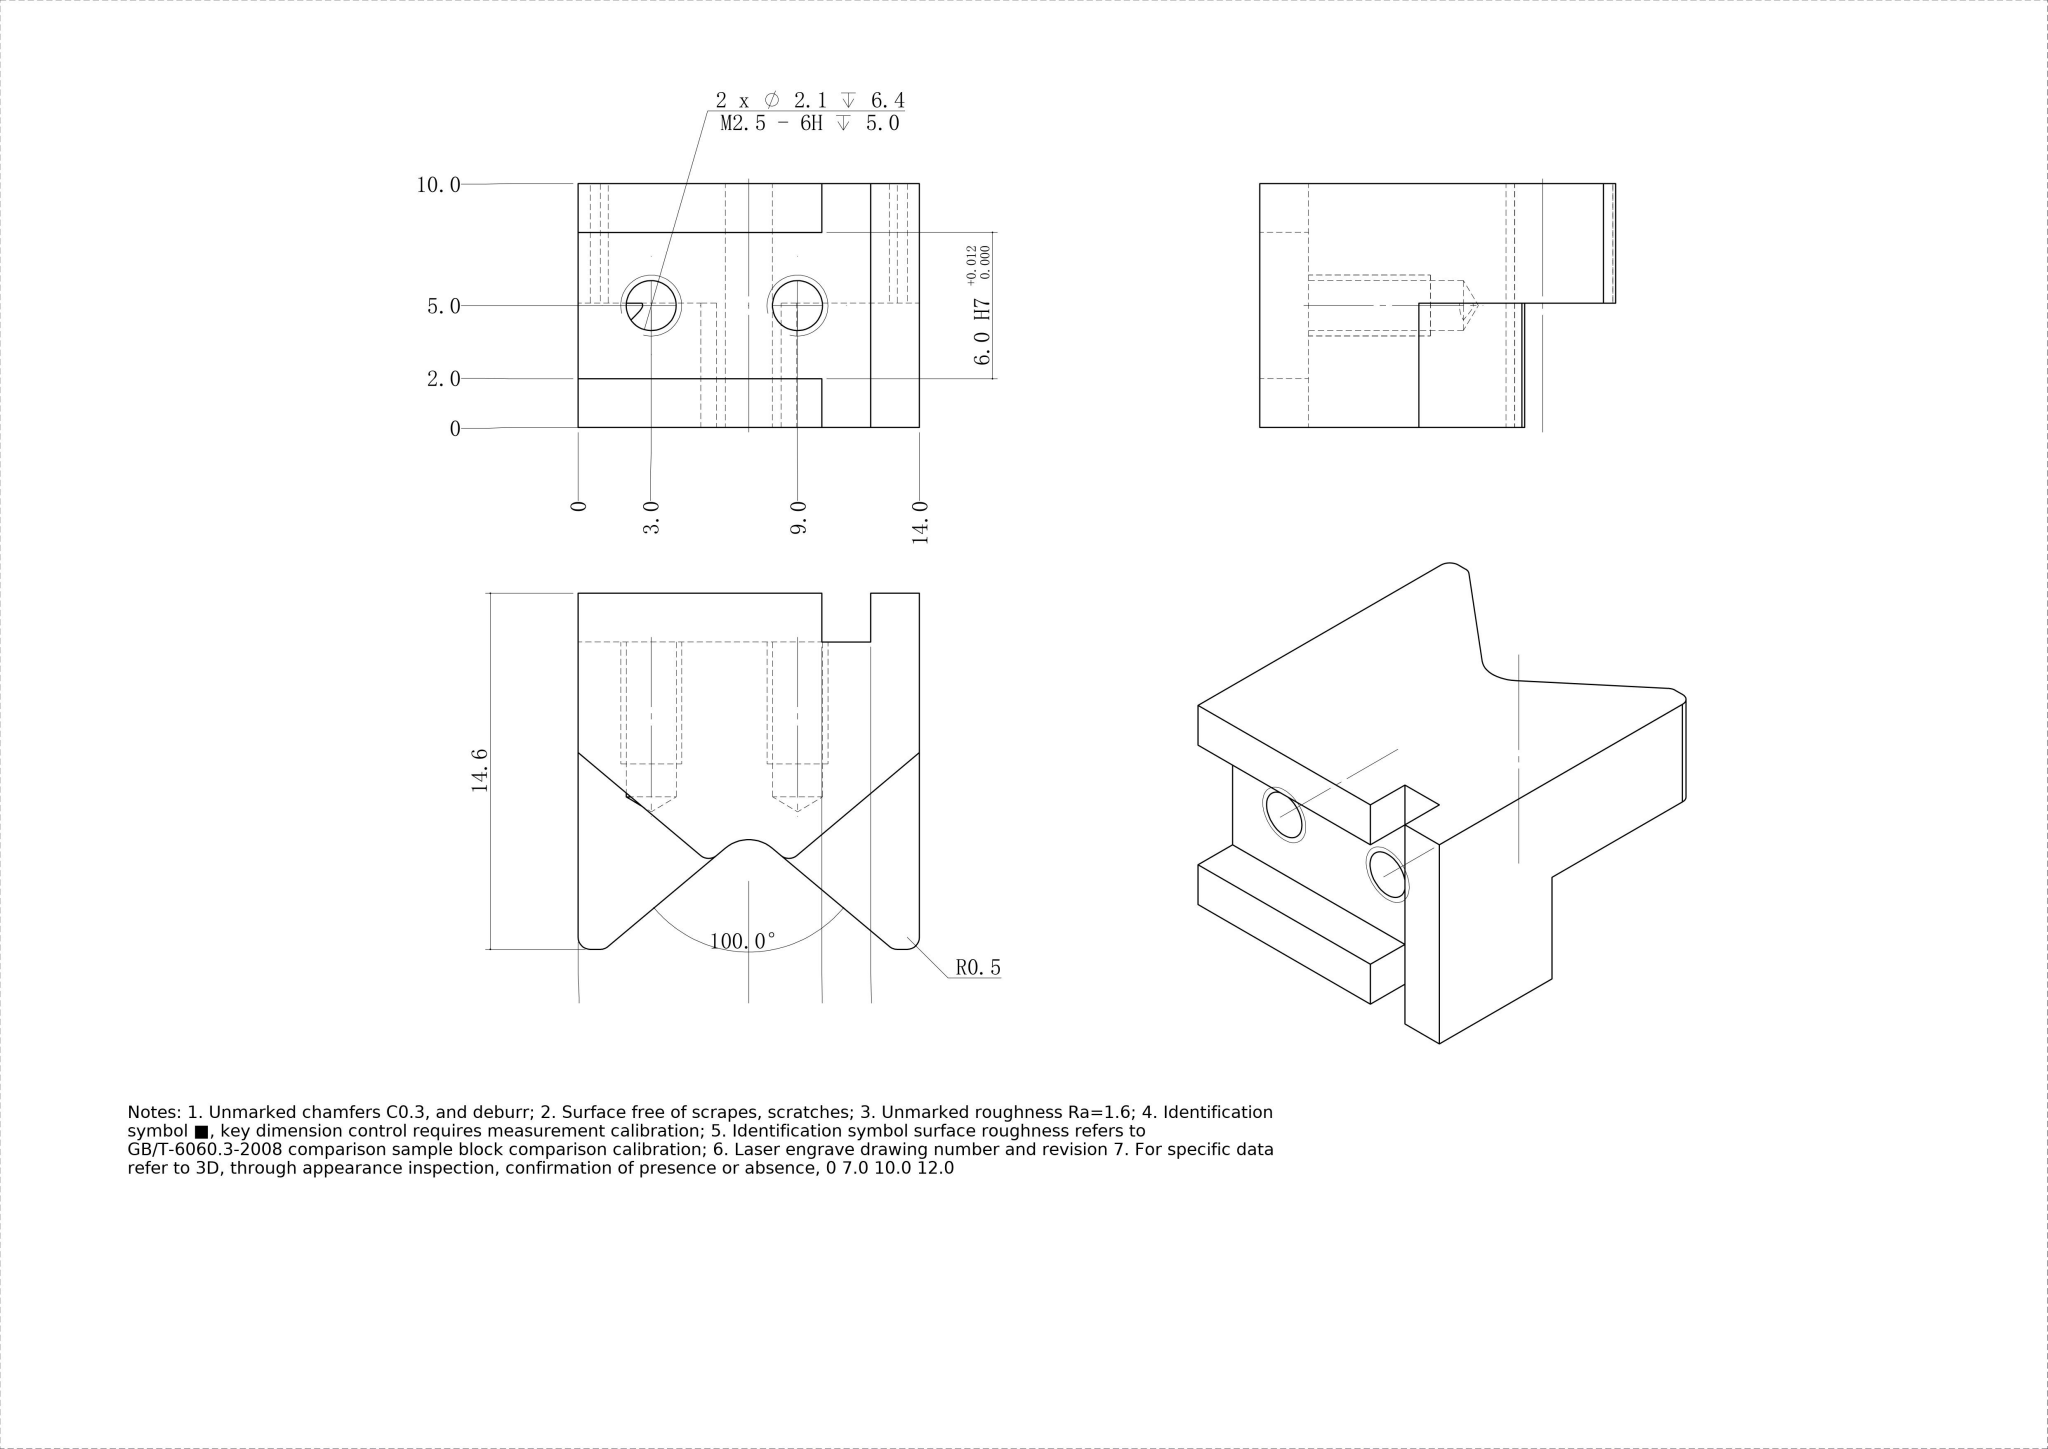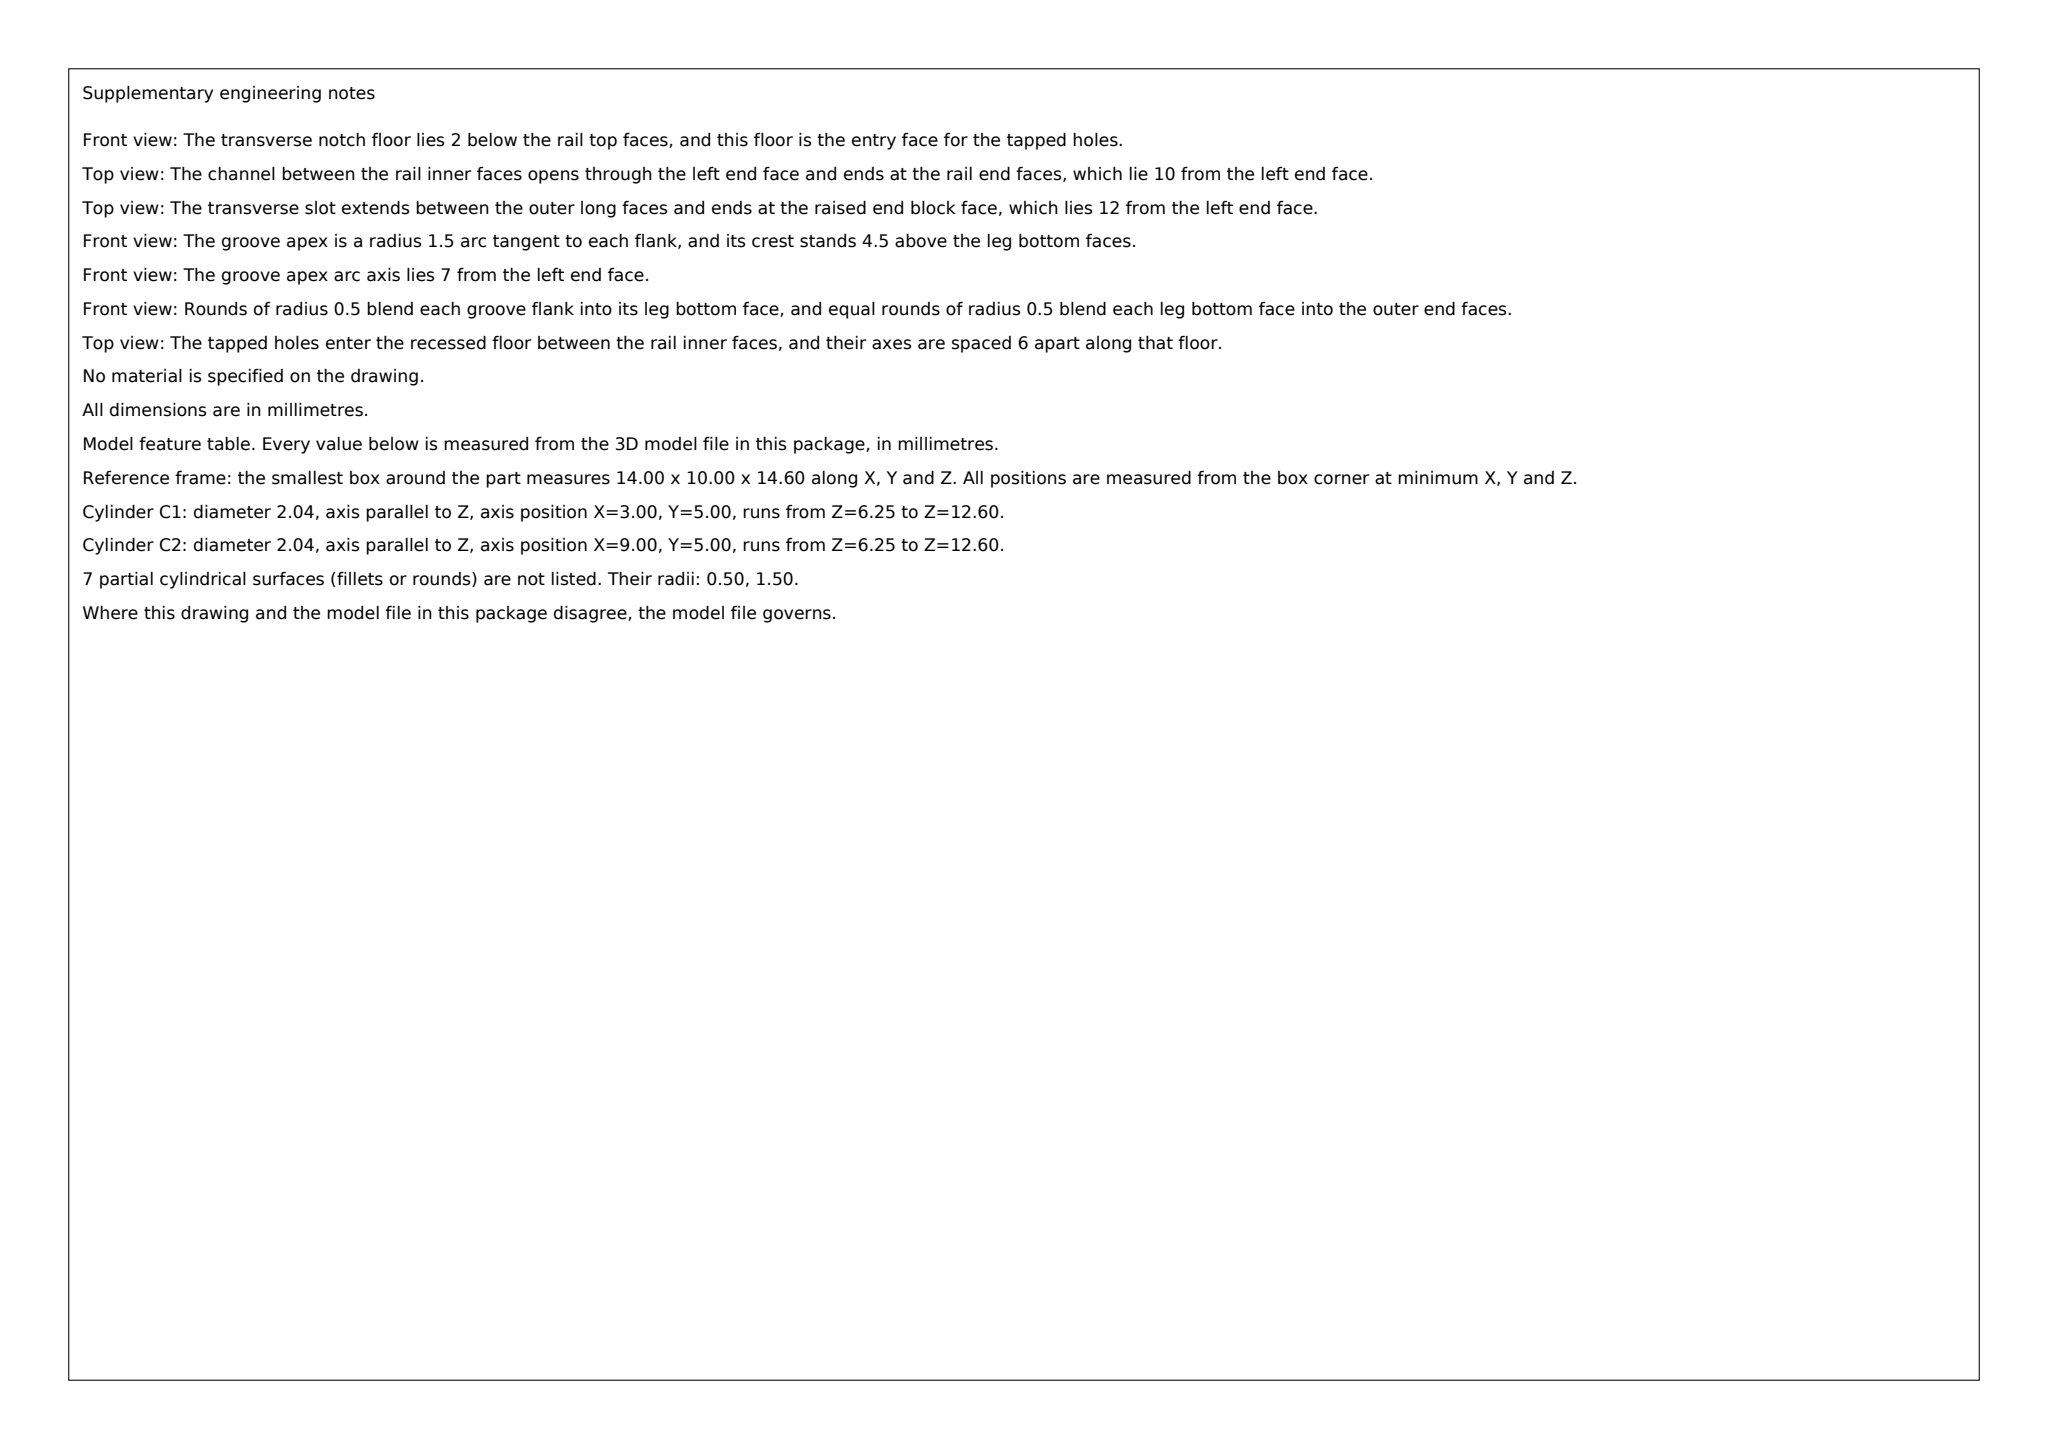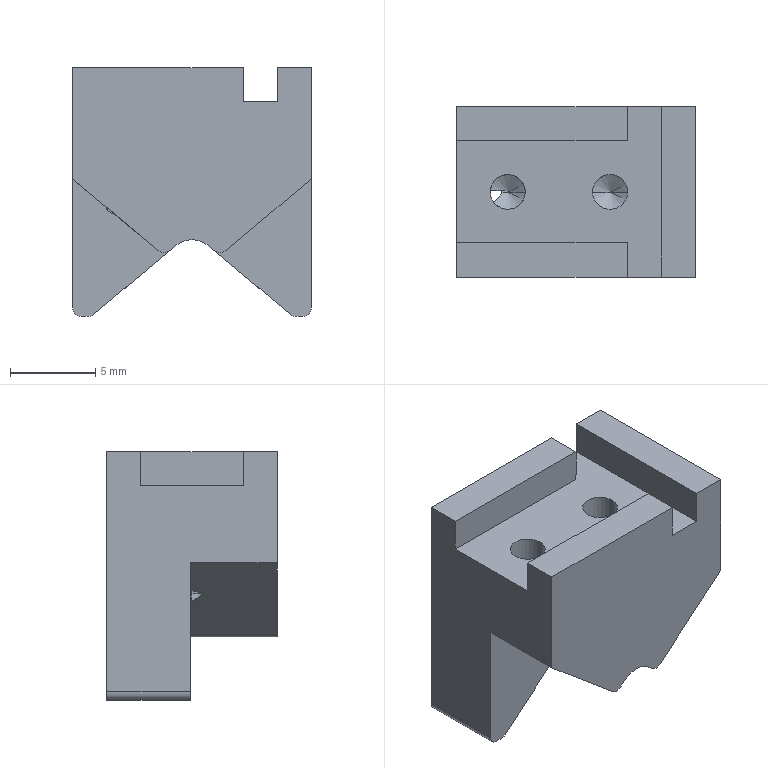Part | SolidWorks | mm | 1 solid | 38 faces | box 14 x 10 x 14.6 mm | volume 1310 mm3 | plane 21 | cylinder 13 | cone 4 | commonest cylinder face diameters 1 x8 2.05 x4 3 x1
Drawing notes:
FRONT VIEW: V-GROOVE / R1.5 CL AT X=7.0 FROM LH END FACE | from the solid: Ø3.0 y-axis cyl at x=7.0, z=3.0; V form centred on same axis
STEP / SHOULDER FACE 10.0 FROM LH END FACE | from the solid: axis_plane normal x, offset 10.0 (count 2)
TOP NOTCH 2.0 DP x 2.0 WIDE; FACE 12.0 FROM LH END FACE | from the solid: x planes at 12.0 and 14.0 (bbox X=14.0); notch depth 2.0 (balloon 1)
SIDE VIEW: RH STEP 2.0 DP; FACE 8.0 FROM FRONT FACE Y=0 | from the solid: y planes at 8.0 and 10.0; bbox Y=10.0
V-GROOVE RUN-OUT FACE 5.1 FROM FRONT FACE Y=0 | from the solid: axis_plane normal y, offset 5.1 (count 2); Ø1.0 y-cyl length 5.1
build123d program:
from build123d import *

# Parameters (mm, degrees)
SKETCH1_2_W             = 14
SKETCH1_2_H             = 10
BOSS_EXTRUDE1_DEPTH     = 7.3
CUT_EXTRUDE2_DEPTH      = 15.223
SKETCH1_W               = 24
SKETCH1_H               = 6
EXTRUDE1_DEPTH          = 2
SKETCH2_W               = 2
SKETCH2_H               = 10
EXTRUDE2_DEPTH          = 2
EXTRUDE3_DEPTH          = 5.1
M2_5_TAPPED_HOLE1_D     = 2.05
M2_5_TAPPED_HOLE1_DEPTH = 6.35
M2_5_TAPPED_HOLE1_TIP   = 0.6159
FILLET1_R               = 0.5


with BuildPart() as part:
    # Sketch1_2 → Boss-Extrude1 (new, symmetric)
    with BuildSketch(Plane.XY):
        Rectangle(SKETCH1_2_W, SKETCH1_2_H)
    extrude(amount=BOSS_EXTRUDE1_DEPTH, both=True)

    # Sketch4 → Cut-Extrude2 (cut, through all)
    with BuildSketch(Plane(origin=(0, -5, 0), x_dir=(-1, 0, 0), z_dir=(0, -1, 0))):
        with BuildLine():
            Line((-5.909, 7.3), (-0.9642, 3.151))
            ThreePointArc((-0.9642, 3.151), (0, 2.8), (0.9642, 3.151))
            Line((0.9642, 3.151), (5.909, 7.3))
            Line((5.909, 7.3), (-5.909, 7.3))
        make_face()
    extrude(amount=-CUT_EXTRUDE2_DEPTH, mode=Mode.SUBTRACT)

    # Sketch1 → Extrude1 (cut)
    with BuildSketch(Plane(origin=(0, 0, 7.3), x_dir=(-1, 0, 0), z_dir=(0, 0, -1))):
        with Locations((7, 0)):
            Rectangle(SKETCH1_W, SKETCH1_H)
    extrude(amount=EXTRUDE1_DEPTH, mode=Mode.SUBTRACT)

    # Sketch2 → Extrude2 (cut)
    with BuildSketch(Plane(origin=(0, 0, 7.3), x_dir=(-1, 0, 0), z_dir=(0, 0, -1))):
        with Locations((-4, 0)):
            Rectangle(SKETCH2_W, SKETCH2_H)
    extrude(amount=EXTRUDE2_DEPTH, mode=Mode.SUBTRACT)

    # Sketch3 → Extrude3 (cut)
    with BuildSketch(Plane.XZ.offset(5)):
        Polygon((7, -7.3), (7, 0.7683), (1.647, -3.724), (5.909, -7.3), align=None)
        Polygon((-5.909, -7.3), (-1.647, -3.724), (-7, 0.7683), (-7, -7.3), align=None)
    extrude(amount=-EXTRUDE3_DEPTH, mode=Mode.SUBTRACT)

    # M2.5 Tapped Hole1
    with Locations(Plane.XY.offset(5.3)):
        with Locations((2, 0), (-4, 0)):
            Hole(M2_5_TAPPED_HOLE1_D / 2, depth=M2_5_TAPPED_HOLE1_DEPTH)
            with Locations((0, 0, -(M2_5_TAPPED_HOLE1_DEPTH + M2_5_TAPPED_HOLE1_TIP / 2))):  # 118° drill point
                Cone(0, M2_5_TAPPED_HOLE1_D / 2, M2_5_TAPPED_HOLE1_TIP, mode=Mode.SUBTRACT)

    # Fillet1
    fillet1_edges = [part.edges().sort_by_distance(p)[0] for p in [
        (5.909, 2.55, -7.3),
        (-5.909, 2.55, -7.3),
        (-7, 2.55, -7.3),
        (7, 2.55, -7.3),
        (1.647, -2.45, -3.724),
        (-1.647, -2.45, -3.724),
    ]]
    fillet(fillet1_edges, radius=FILLET1_R)


solid = part.part